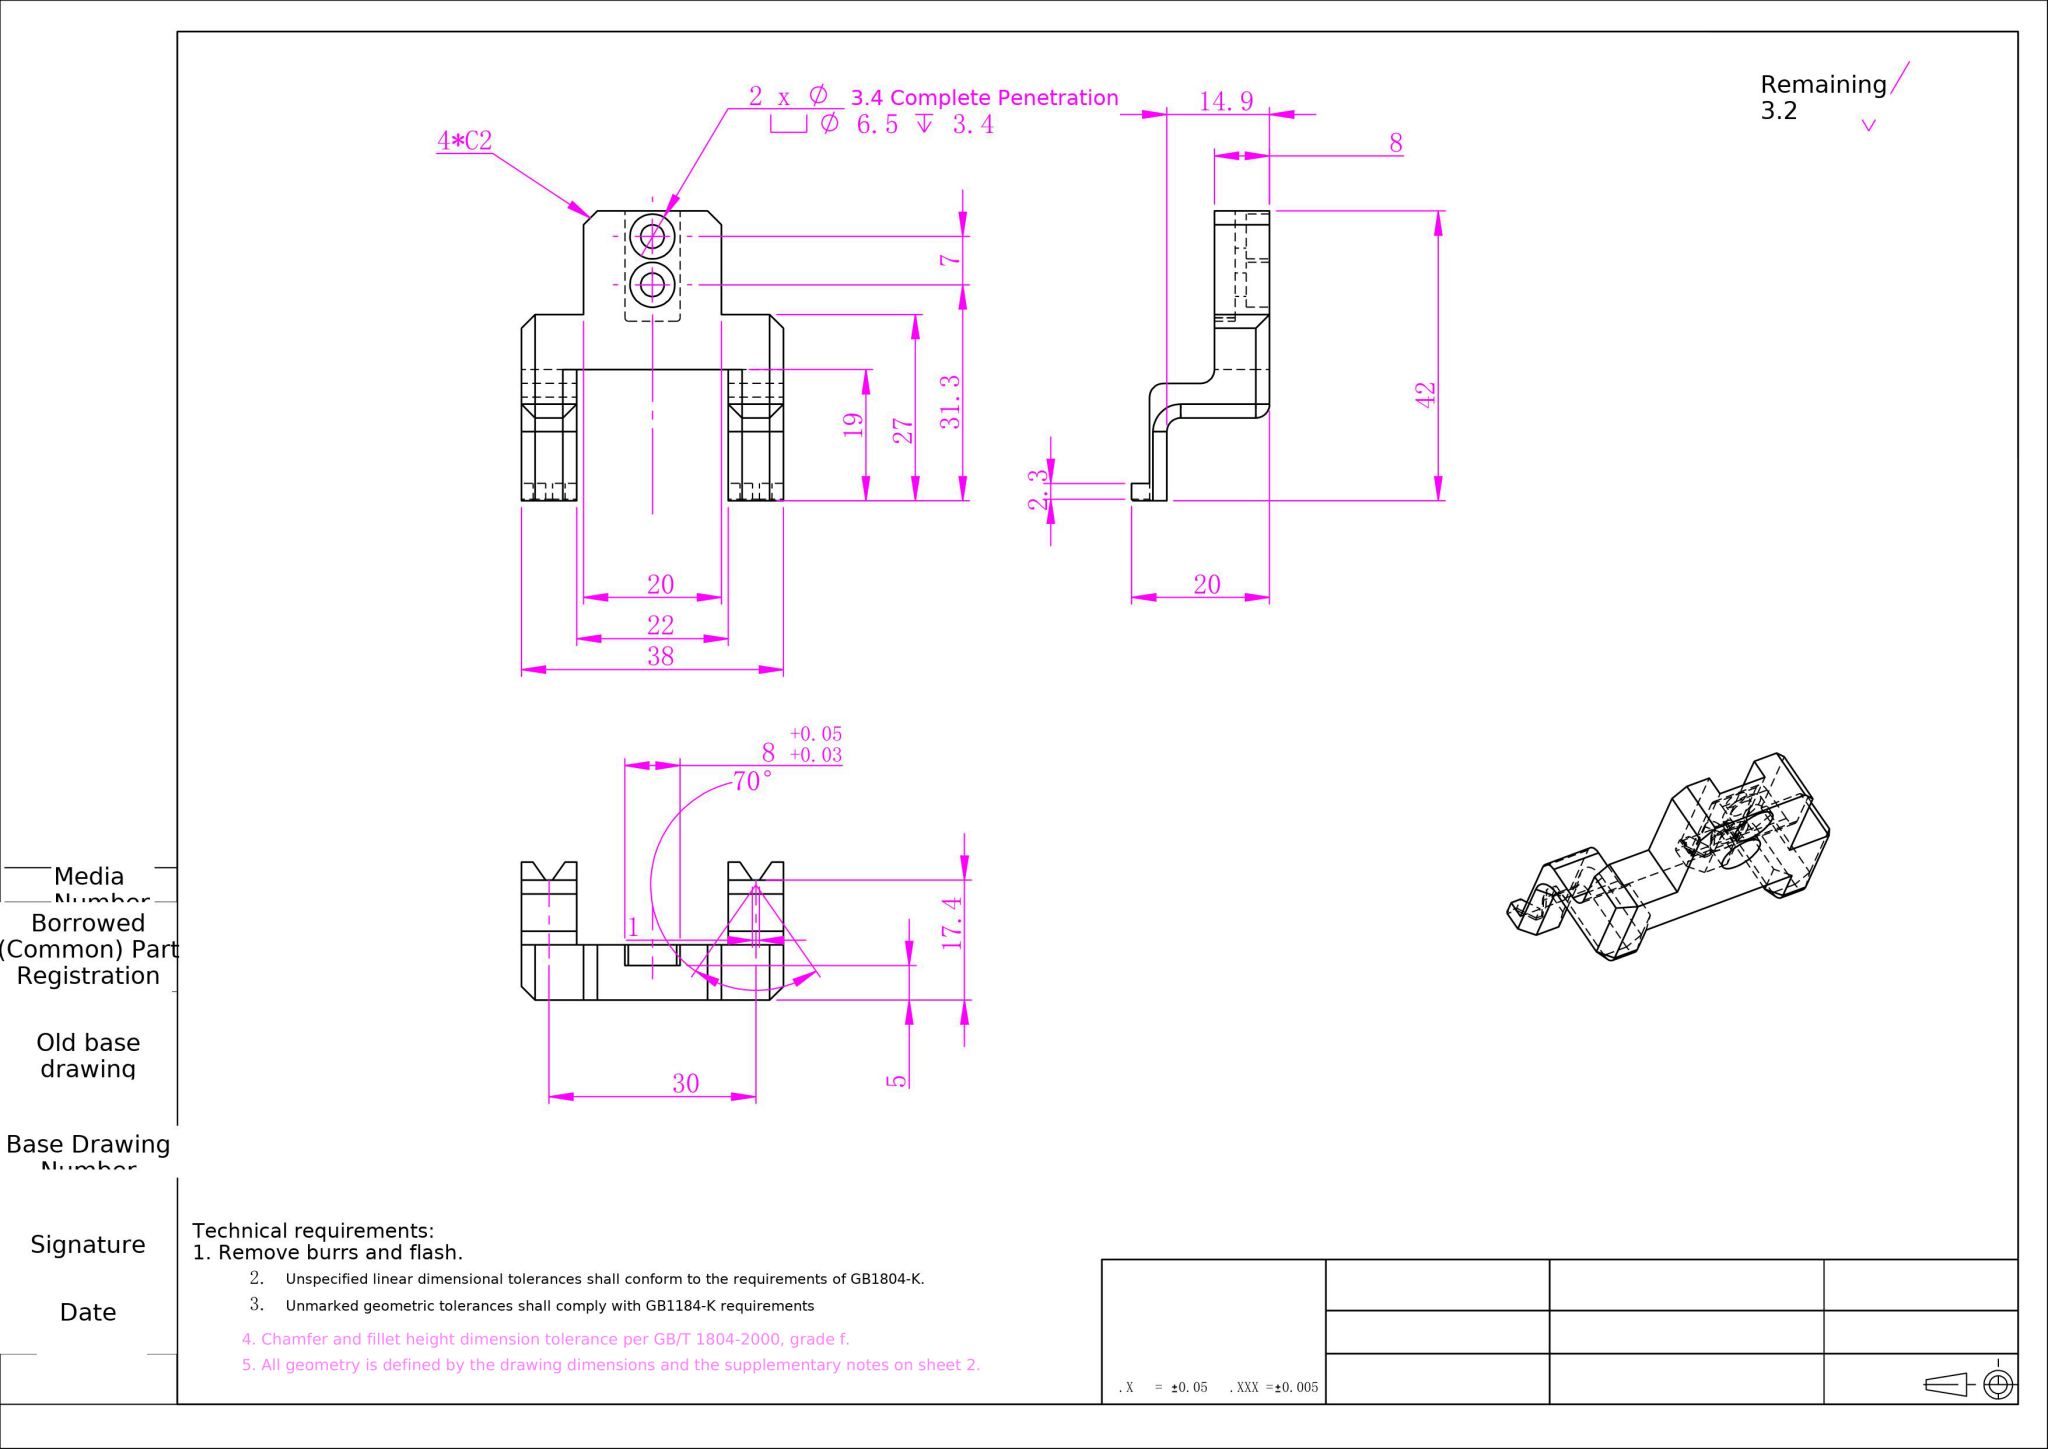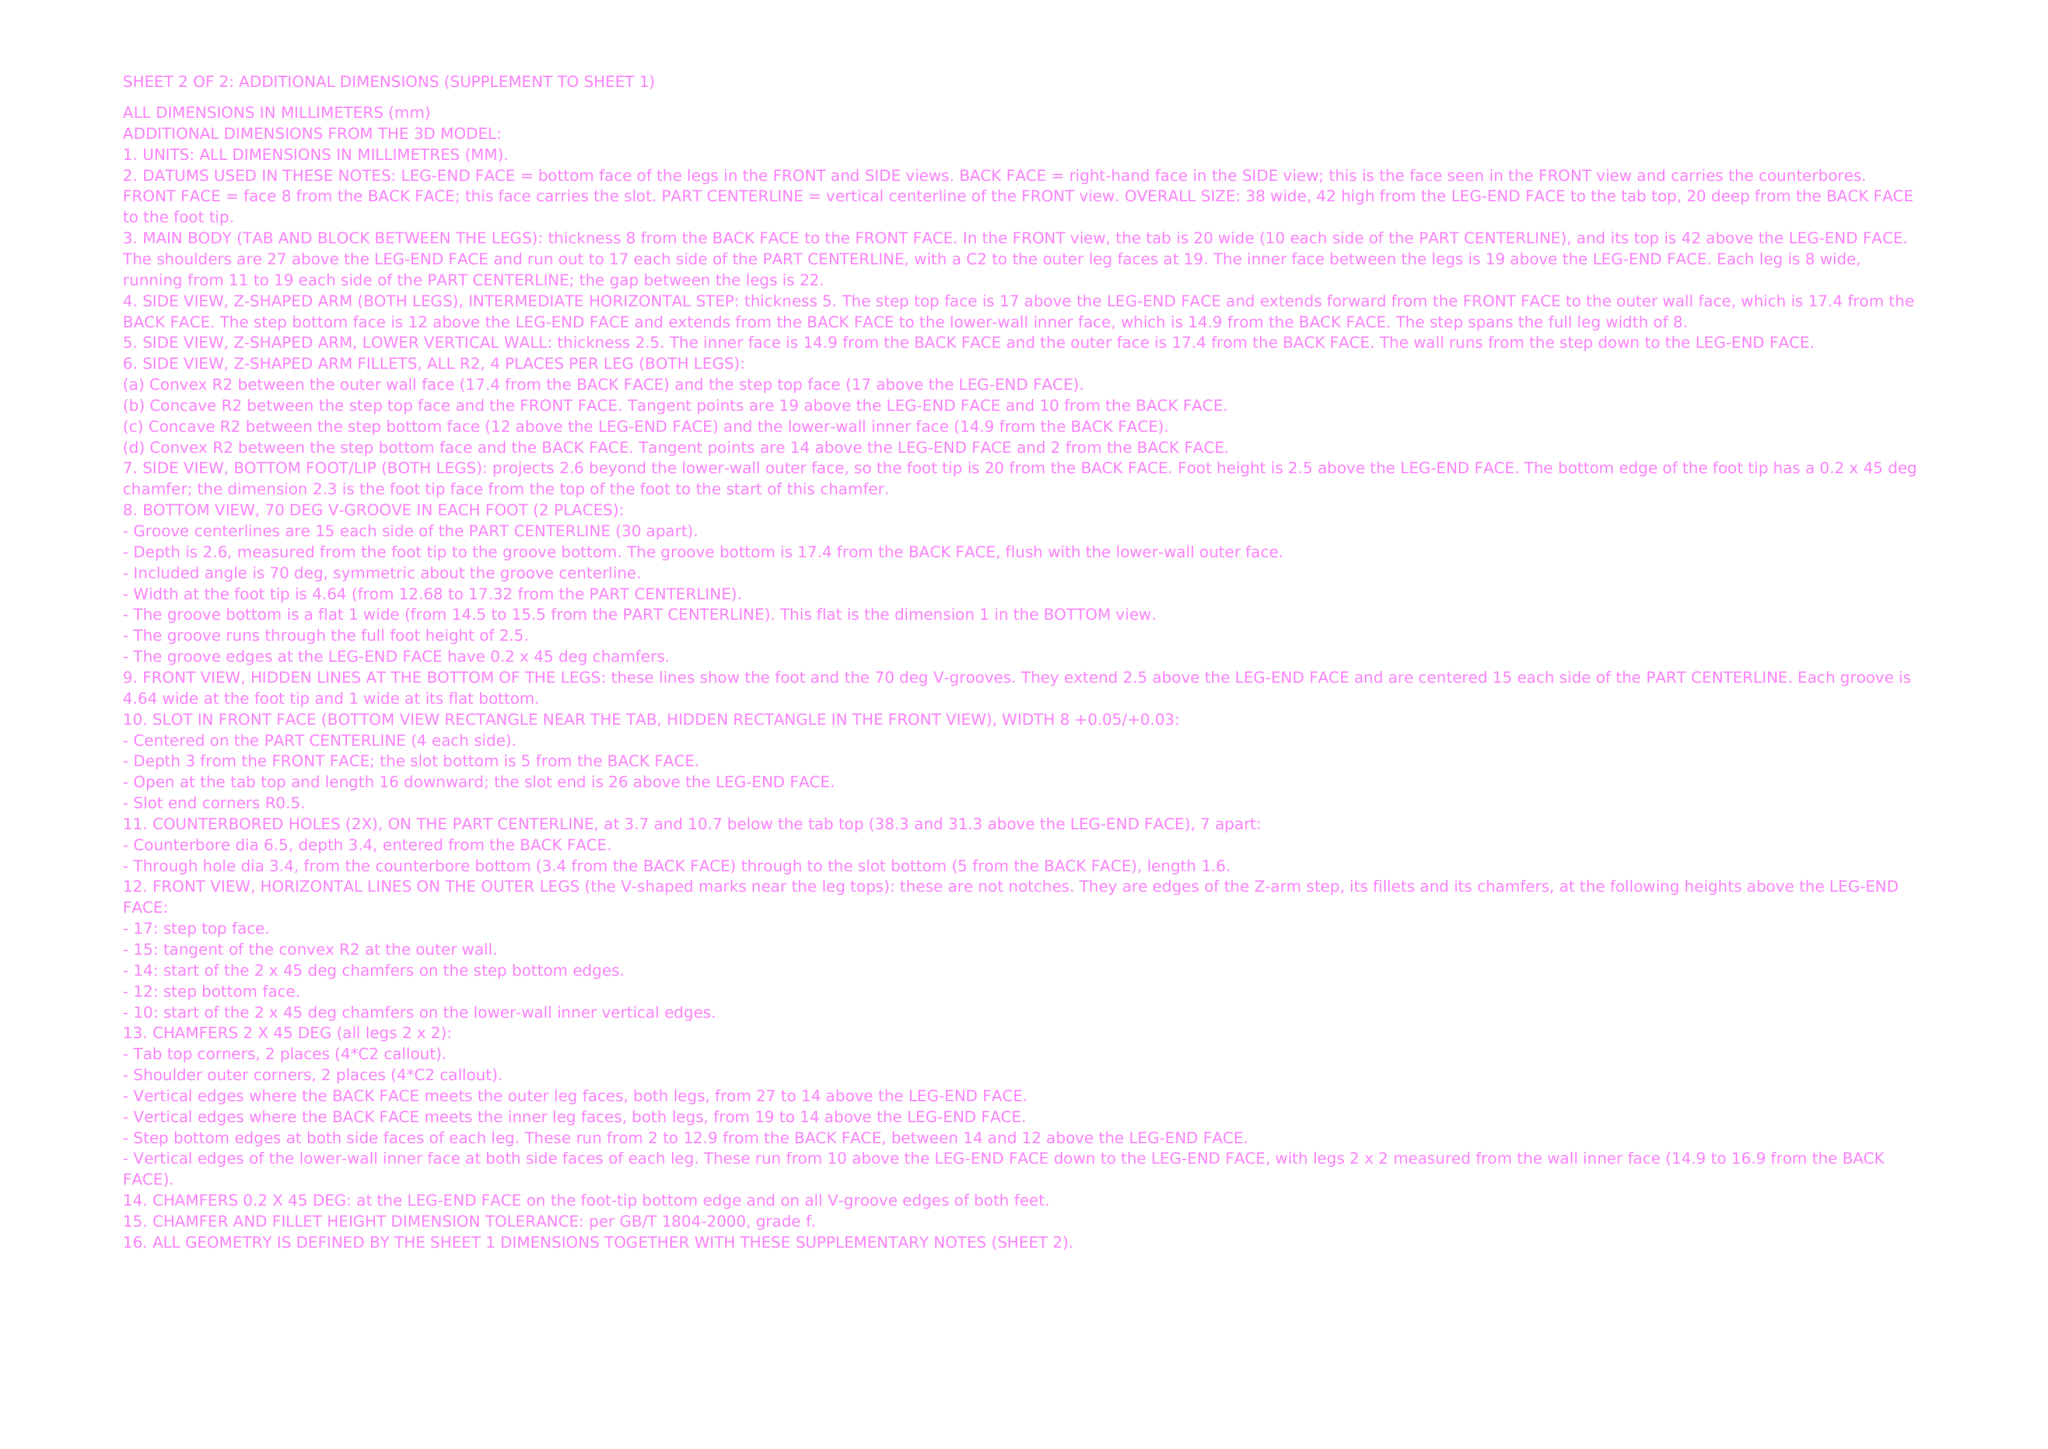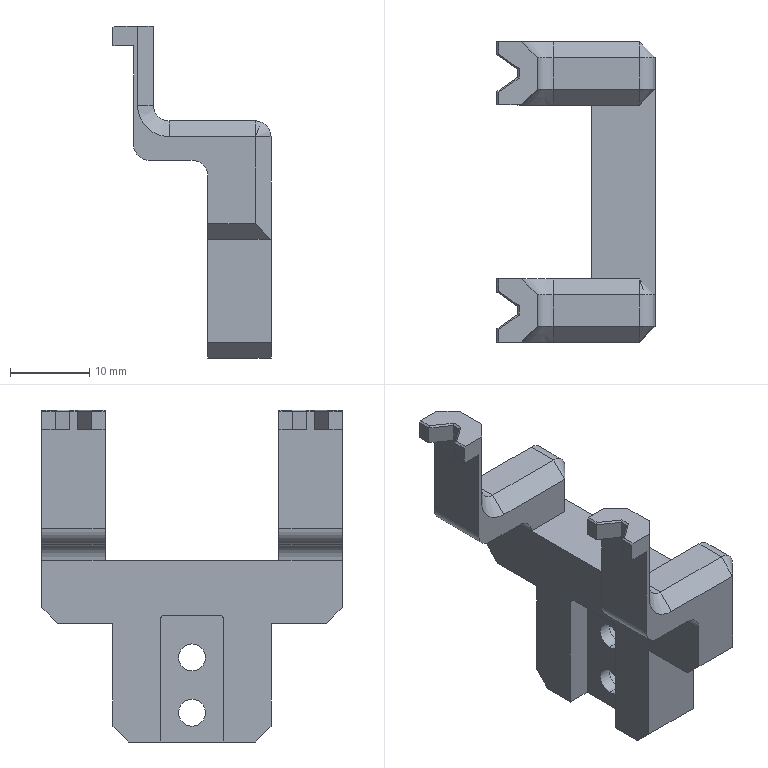Part | NX | mm | 1 solid | 92 faces | box 20 x 38 x 42 mm | volume 6040 mm3 | plane 66 | cylinder 18 | cone 8 | commonest cylinder face diameters 4 x8 6.5 x4 3.4 x4 1 x2